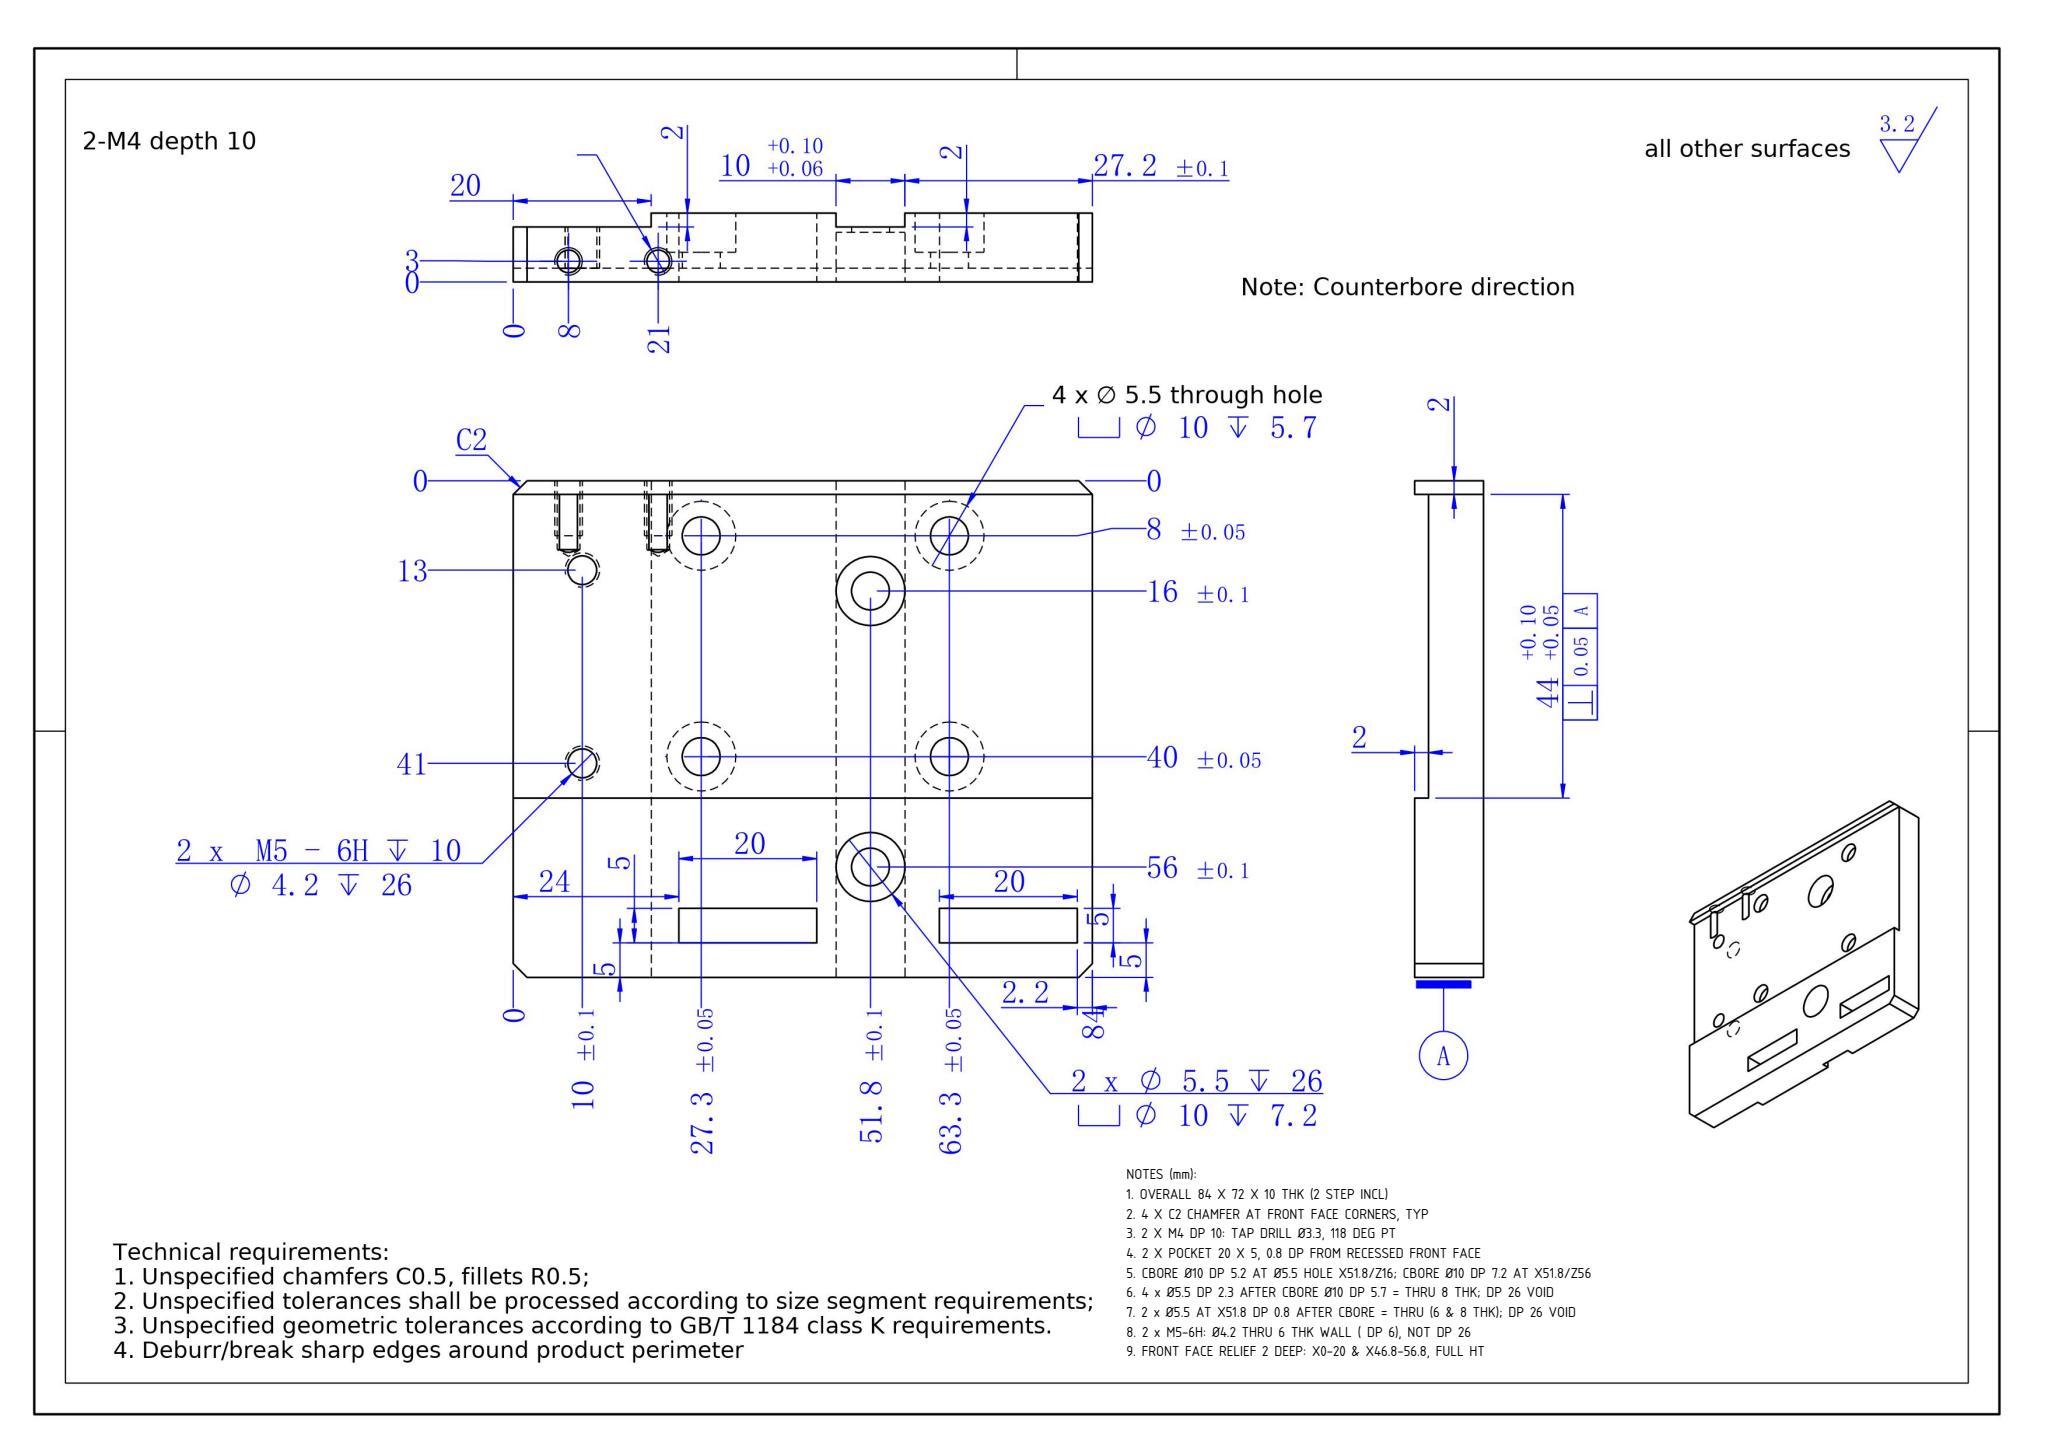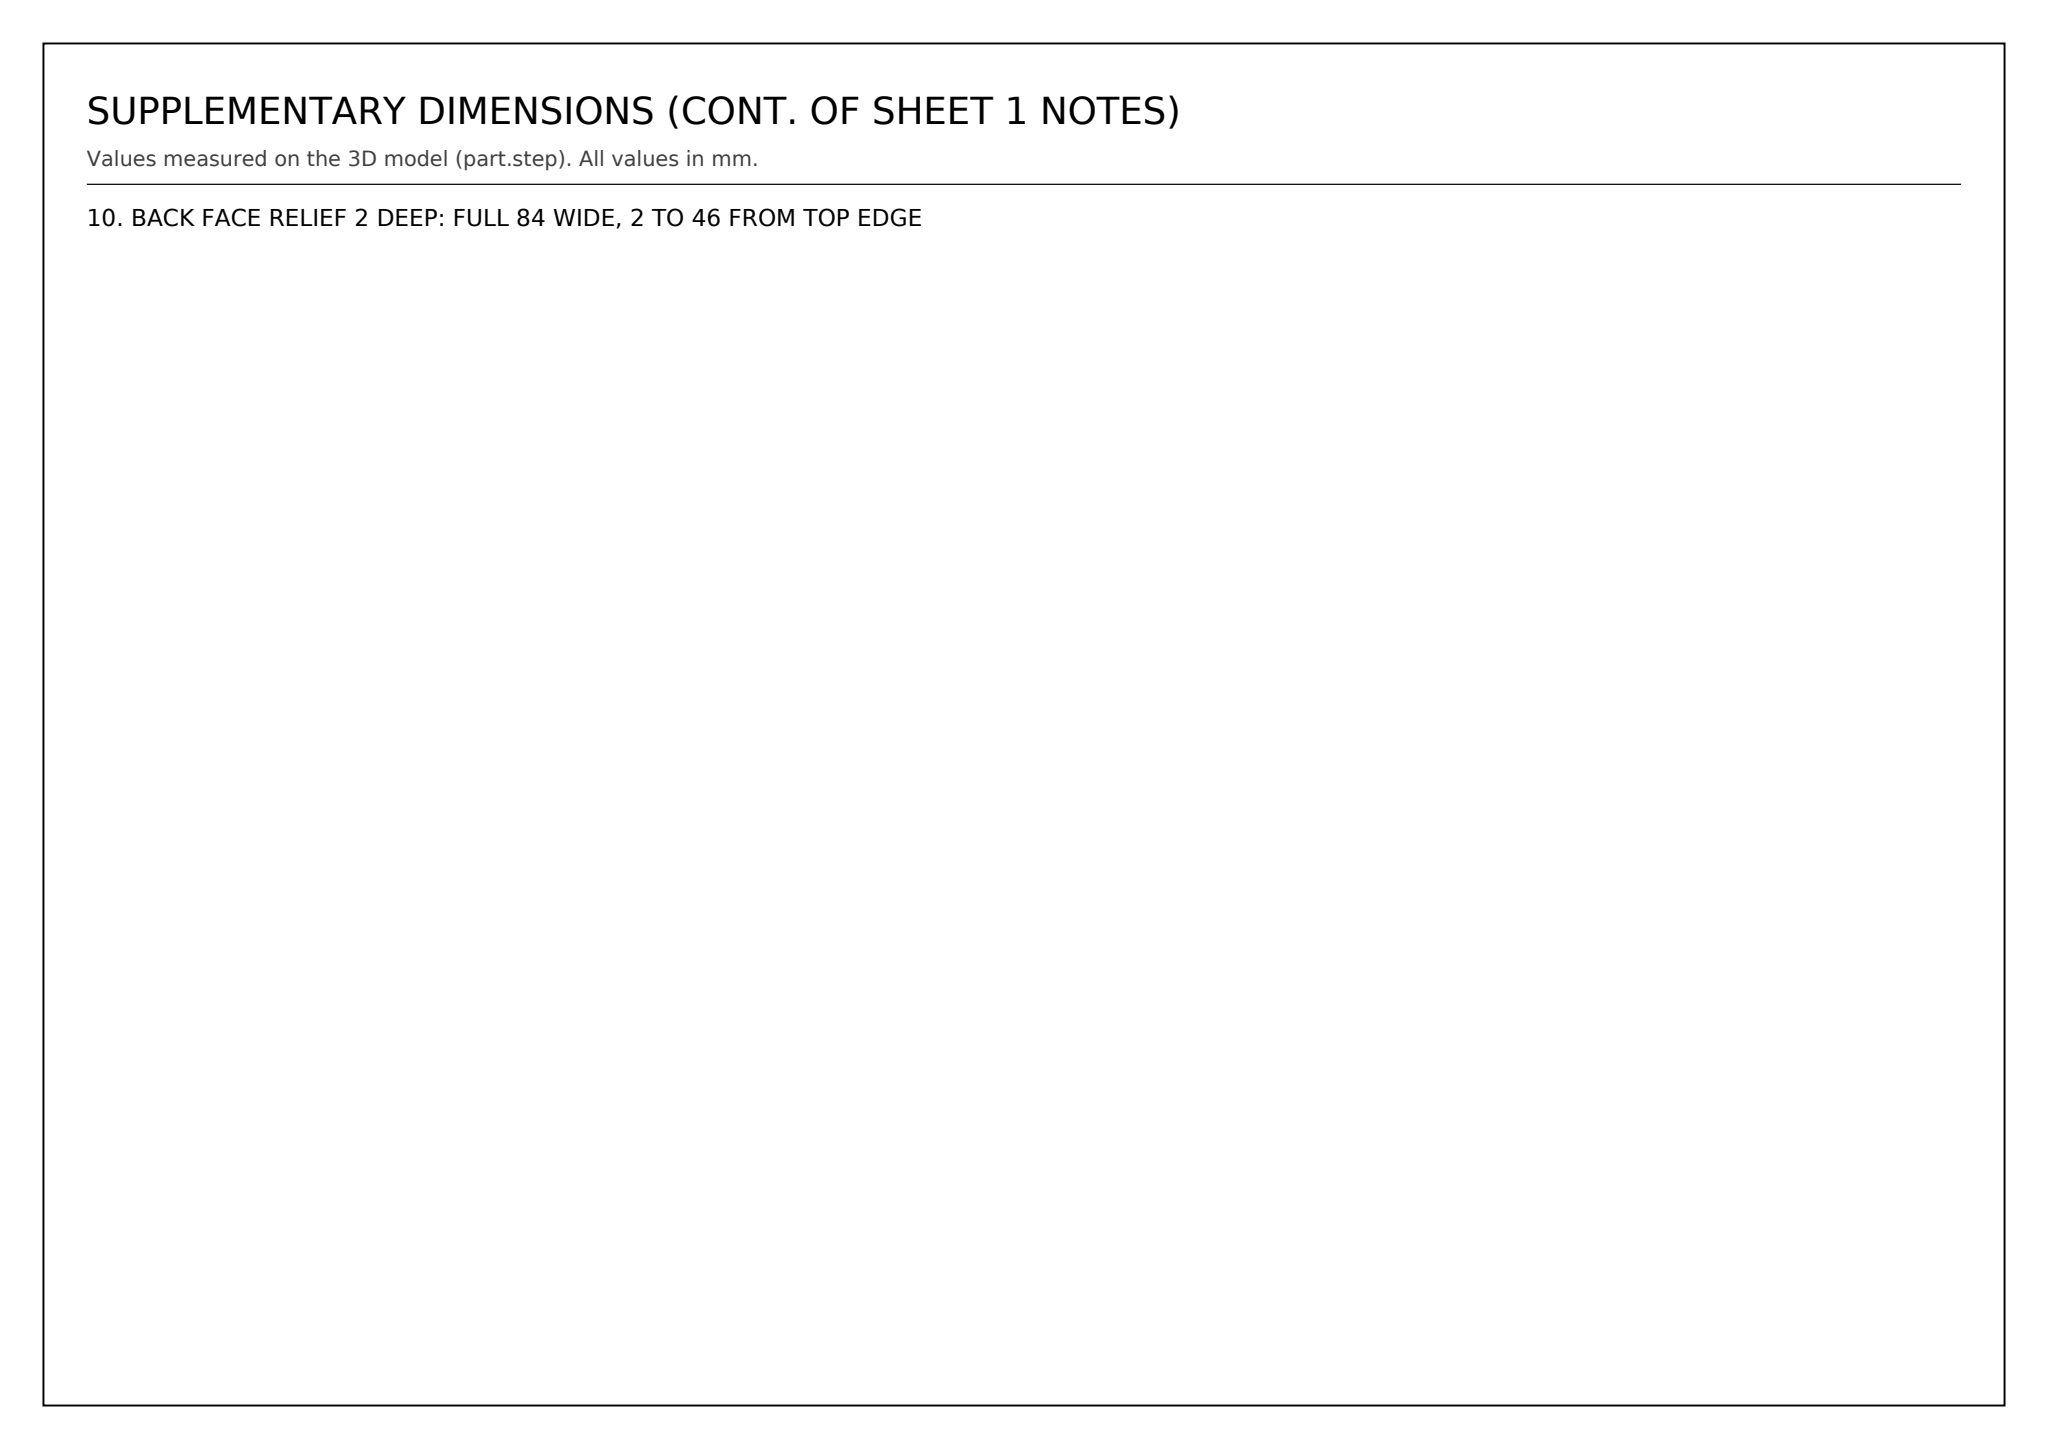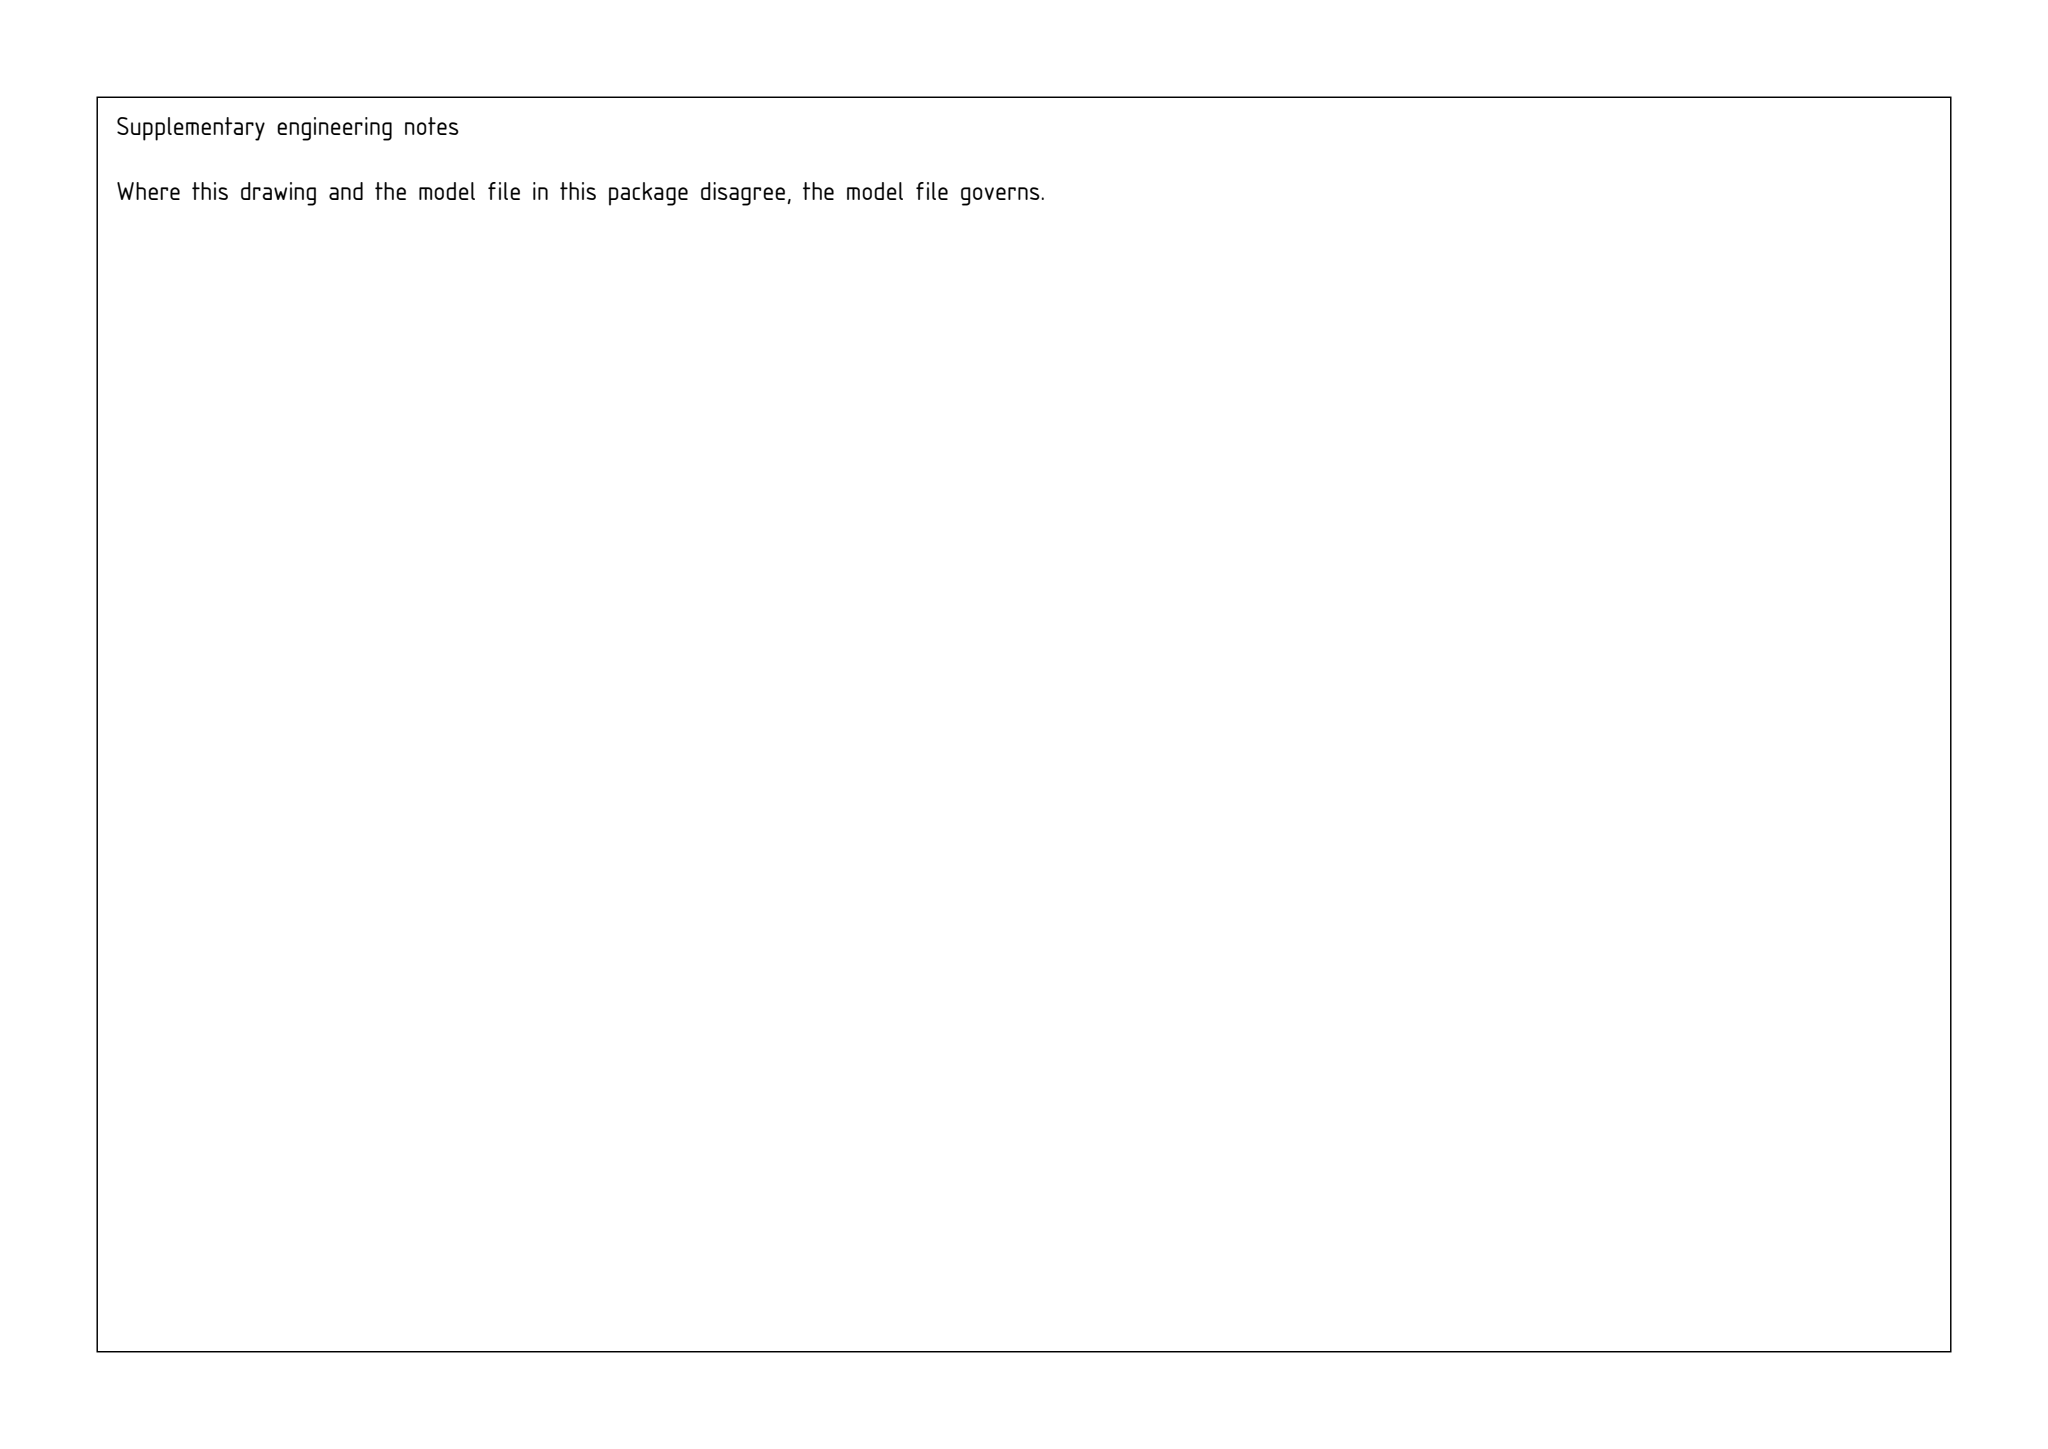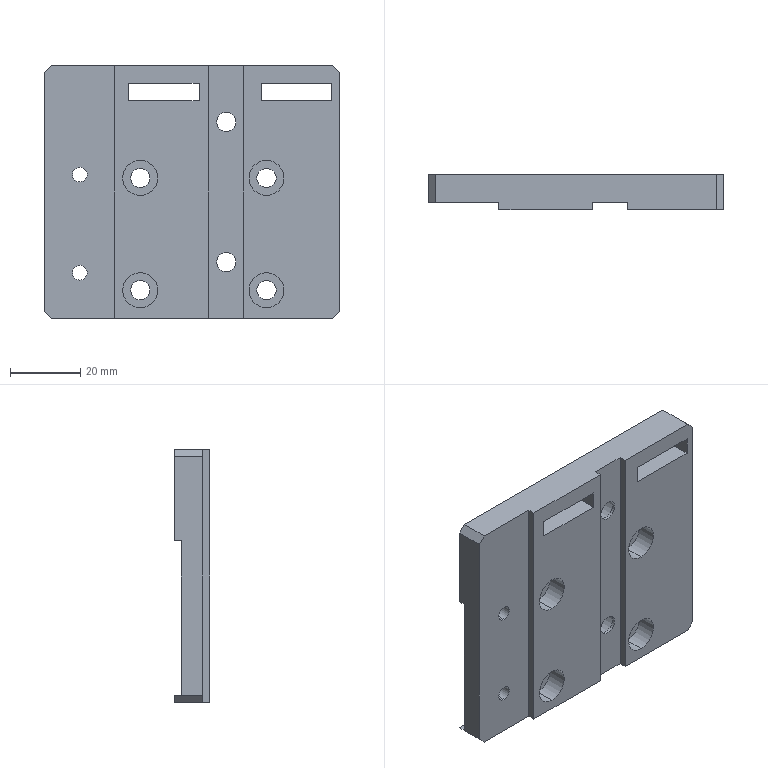Part | SolidWorks | mm | 1 solid | 70 faces | box 84 x 10 x 72 mm | volume 43351 mm3 | plane 34 | cylinder 32 | cone 4 | commonest cylinder face diameters 10 x12 5.5 x12 4.2 x4 3.3 x4
Drawing notes:
OVERALL 84 X 72 X 10 THK (2 STEP INCL) | from the solid: bbox_xyz [84.001,10.001,72.001]; y planes 0.0/2.0/10.0; z planes 0.0/72.0
4 X C2 CHAMFER AT FRONT FACE CORNERS, TYP | from the solid: 84 x 72 front face, all 4 corners cut 2 x 2 at 45 deg; only one C2 noted on sheet 1
2 X M4 DP 10: TAP DRILL Ø3.3, 118 DEG PT | from the solid: Ø3.3 z-axis cyls at (8,7) and (21,7), lg 10; cones 118 deg ref dia 3.3
2 X POCKET 20 X 5, 0.8 DP FROM RECESSED FRONT FACE | from the solid: x planes 24/44 & 61.8/81.8 (20 lg), z planes 62/67 (5 hi), flr y=2.8 vs face y=2.0
CBORE Ø10 DP 5.2 AT Ø5.5 HOLE X51.8/Z16; CBORE Ø10 DP 7.2 AT X51.8/Z56 | from the solid: cyl Ø10 y-axis at (51.8,16) len 5.2; Ø10 y-axis at (51.8,56) len 7.2
4 x Ø5.5 DP 2.3 AFTER CBORE Ø10 DP 5.7 = THRU 8 THK; DP 26 VOID | from the solid: Ø5.5 y-axis at (27.25,8),(27.25,40),(63.25,8),(63.25,40) len 2.3 + Ø10 cbore 5.7 = 8 = wall y0-y8
2 x Ø5.5 AT X51.8 DP 0.8 AFTER CBORE = THRU (6 & 8 THK); DP 26 VOID | from the solid: Ø5.5 y-axis at (51.8,16) & (51.8,56) len 0.8; 5.2+0.8=6 thru y2-y8, 7.2+0.8=8 thru y2-y10
2 x M5-6H: Ø4.2 THRU 6 THK WALL ( DP 6), NOT DP 26 | from the solid: Ø4.2 y-axis at (10,12.97) & (10,40.97) len 6.0, from y=2 recessed face to y=8
FRONT FACE RELIEF 2 DEEP: X0-20 & X46.8-56.8, FULL HT | from the solid: y-planes 0 (2 faces) & 2 (2 faces); x-planes 20, 46.8, 56.8
BACK FACE RELIEF 2 DEEP: FULL 84 WIDE, 2 TO 46 FROM TOP EDGE | from the solid: single y=8 plane; z-planes 2 and 46, 46-2=44 (44 +0.10/+0.05 dim)
build123d program:
from build123d import *

# Parameters (mm, degrees)
SKETCH1_W                                         = 84
SKETCH1_H                                         = 72
BOSS_EXTRUDE1_DEPTH                               = 10
CHAMFER1_SIZE                                     = 2
SKETCH12_W                                        = 44
SKETCH12_H                                        = 2
CUT_EXTRUDE3_DEPTH                                = 112.086
HOLE_SIZE_ACCORDING_TO_HEXAGON_SOCKET_D           = 5.5
HOLE_SIZE_ACCORDING_TO_HEXAGON_SOCKET_CBORE_D     = 10
HOLE_SIZE_ACCORDING_TO_HEXAGON_SOCKET_CBORE_DEPTH = 5.7
M4_TAPPED_HOLE2_D                                 = 3.3
M4_TAPPED_HOLE2_DEPTH                             = 10
M4_TAPPED_HOLE2_TIP                               = 0.9914
SKETCH22_W                                        = 10
SKETCH22_H                                        = 2
CUT_EXTRUDE4_DEPTH                                = 112.086
HOLE_SIZE_ACCORDING_TO_HEXAGON_SOC_2_D            = 5.5
HOLE_SIZE_ACCORDING_TO_HEXAGON_SOC_2_DEPTH        = 26
HOLE_SIZE_ACCORDING_TO_HEXAGON_SOC_2_CBORE_D      = 10
HOLE_SIZE_ACCORDING_TO_HEXAGON_SOC_2_CBORE_DEPTH  = 7.2
HOLE_SIZE_ACCORDING_TO_HEXAGON_SOC_2_TIP          = 1.652
SKETCH27_W                                        = 20
SKETCH27_H                                        = 72
CUT_EXTRUDE5_DEPTH                                = 2
M5_TAPPED_HOLE1_D                                 = 4.2
M5_TAPPED_HOLE1_DEPTH                             = 26
M5_TAPPED_HOLE1_TIP                               = 1.262
SKETCH30_W                                        = 20
SKETCH30_H                                        = 5
CUT_EXTRUDE6_DEPTH                                = 10


with BuildPart() as part:
    # Sketch1 → Boss-Extrude1 (new body)
    with BuildSketch(Plane(origin=(0, 0, 0), x_dir=(1, 0, 0), z_dir=(0, 1, 0))):
        with Locations((42, 36)):
            Rectangle(SKETCH1_W, SKETCH1_H)
    extrude(amount=BOSS_EXTRUDE1_DEPTH)

    # Chamfer1
    chamfer1_edges = [part.edges().sort_by_distance(p)[0] for p in [
        (0, 5, -72),
        (84, 5, -72),
        (84, 5, 0),
        (0, 5, 0),
    ]]
    chamfer(chamfer1_edges, length=CHAMFER1_SIZE)

    # Sketch12 → Cut-Extrude3 (cut, through all)
    with BuildSketch(Plane.ZY):
        with Locations((-48, 9)):
            Rectangle(SKETCH12_W, SKETCH12_H)
    extrude(amount=-CUT_EXTRUDE3_DEPTH, mode=Mode.SUBTRACT)

    # Hole Size _according to_ Hexagon Socket (through all)
    with Locations(Plane(origin=(0, 0, 0), x_dir=(-1, 0, 0), z_dir=(0, -1, 0))):
        with Locations((-63.25, 64), (-27.25, 64), (-27.25, 32), (-63.25, 32)):
            CounterBoreHole(HOLE_SIZE_ACCORDING_TO_HEXAGON_SOCKET_D / 2, HOLE_SIZE_ACCORDING_TO_HEXAGON_SOCKET_CBORE_D / 2, HOLE_SIZE_ACCORDING_TO_HEXAGON_SOCKET_CBORE_DEPTH)

    # M4 Tapped Hole2
    with Locations(Plane(origin=(0, 0, -72), x_dir=(-1, 0, 0), z_dir=(0, 0, -1))):
        with Locations((-21, 7), (-8, 7)):
            Hole(M4_TAPPED_HOLE2_D / 2, depth=M4_TAPPED_HOLE2_DEPTH)
            with Locations((0, 0, -(M4_TAPPED_HOLE2_DEPTH + M4_TAPPED_HOLE2_TIP / 2))):  # 118° drill point
                Cone(0, M4_TAPPED_HOLE2_D / 2, M4_TAPPED_HOLE2_TIP, mode=Mode.SUBTRACT)

    # Sketch22 → Cut-Extrude4 (cut, through all)
    with BuildSketch(Plane(origin=(0, 0, -72), x_dir=(-1, 0, 0), z_dir=(0, 0, -1))):
        with Locations((-51.8, 1)):
            Rectangle(SKETCH22_W, SKETCH22_H)
    extrude(amount=-CUT_EXTRUDE4_DEPTH, mode=Mode.SUBTRACT)

    # Hole Size _according to_ Hexagon Soc 2
    with Locations(Plane(origin=(0, 10, 0), x_dir=(1, 0, 0), z_dir=(0, 1, 0))):
        with Locations((51.8, 16), (51.8, 56)):
            CounterBoreHole(HOLE_SIZE_ACCORDING_TO_HEXAGON_SOC_2_D / 2, HOLE_SIZE_ACCORDING_TO_HEXAGON_SOC_2_CBORE_D / 2, HOLE_SIZE_ACCORDING_TO_HEXAGON_SOC_2_CBORE_DEPTH, depth=HOLE_SIZE_ACCORDING_TO_HEXAGON_SOC_2_DEPTH)
            with Locations((0, 0, -(HOLE_SIZE_ACCORDING_TO_HEXAGON_SOC_2_DEPTH + HOLE_SIZE_ACCORDING_TO_HEXAGON_SOC_2_TIP / 2))):  # 118° drill point
                Cone(0, HOLE_SIZE_ACCORDING_TO_HEXAGON_SOC_2_D / 2, HOLE_SIZE_ACCORDING_TO_HEXAGON_SOC_2_TIP, mode=Mode.SUBTRACT)

    # Sketch27 → Cut-Extrude5 (cut)
    with BuildSketch(Plane.XZ):
        with Locations((10, -36)):
            Rectangle(SKETCH27_W, SKETCH27_H)
    extrude(amount=-CUT_EXTRUDE5_DEPTH, mode=Mode.SUBTRACT)

    # M5 Tapped Hole1
    with Locations(Plane(origin=(0, 0, 0), x_dir=(-1, 0, 0), z_dir=(0, -1, 0))):
        with Locations((-10, 59.03), (-10, 31.03)):
            Hole(M5_TAPPED_HOLE1_D / 2, depth=M5_TAPPED_HOLE1_DEPTH)
            with Locations((0, 0, -(M5_TAPPED_HOLE1_DEPTH + M5_TAPPED_HOLE1_TIP / 2))):  # 118° drill point
                Cone(0, M5_TAPPED_HOLE1_D / 2, M5_TAPPED_HOLE1_TIP, mode=Mode.SUBTRACT)

    # Sketch30 → Cut-Extrude6 (cut)
    with BuildSketch(Plane.XZ):
        with Locations((34, -7.5)):
            Rectangle(SKETCH30_W, SKETCH30_H)
        with Locations((71.8, -7.5)):
            Rectangle(SKETCH30_W, SKETCH30_H)
    extrude(amount=-CUT_EXTRUDE6_DEPTH, mode=Mode.SUBTRACT)


solid = part.part